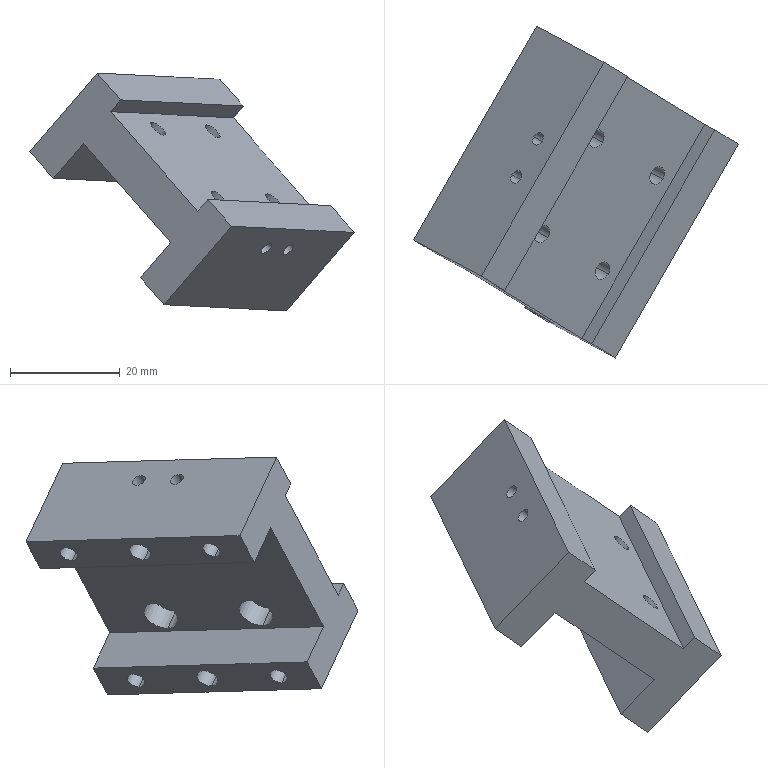Component | SolidWorks | 1z0-123-1 | 1 solid | 74 faces | box 59.17 x 60.52 x 43.37 mm | volume 20475 mm3 | cylinder 36 | cone 20 | plane 18 | commonest cylinder face diameters 2.5 x8 3.3 x8 6.5 x8 3.4 x8 4 x4
build123d program:
from build123d import *

# Parameters (mm, degrees)
SKETCH1_W                                       = 40
SKETCH1_H                                       = 45
BOSS_EXTRUDE1_DEPTH                             = 20
SKETCH2_W                                       = 26
SKETCH2_H                                       = 45
CUT_EXTRUDE1_DEPTH                              = 3
M3_HEX_SOCKET_HEAD_CAP_SCREW_CBORE1_D           = 3.4
M3_HEX_SOCKET_HEAD_CAP_SCREW_CBORE1_CBORE_D     = 6.5
M3_HEX_SOCKET_HEAD_CAP_SCREW_CBORE1_CBORE_DEPTH = 13.4
SKETCH5_W                                       = 26
SKETCH5_H                                       = 18
CUT_EXTRUDE2_DEPTH                              = 54.151
M4_TAPPED_HOLE1_D                               = 3.3
M4_TAPPED_HOLE1_DEPTH                           = 10.1
M4_TAPPED_HOLE1_TIP                             = 0.9914
SIZE_MM_DOWEL_PIN_HOLE1_D                       = 4
SIZE_MM_DOWEL_PIN_HOLE1_DEPTH                   = 10
SIZE_MM_DOWEL_PIN_HOLE1_TIP                     = 1.202
M3_TAPPED_HOLE1_AT_2_COUNT                      = 2
M3_TAPPED_HOLE1_AT_2_PITCH                      = 8


with BuildPart() as part:
    # Sketch1 → Boss-Extrude1 (new body)
    with BuildSketch(Plane.XY):
        Rectangle(SKETCH1_W, SKETCH1_H)
    extrude(amount=BOSS_EXTRUDE1_DEPTH)

    # Sketch2 → Cut-Extrude1 (cut)
    with BuildSketch(Plane(origin=(0, 0, 0), x_dir=(-1, 0, 0), z_dir=(0, 0, -1))):
        Rectangle(SKETCH2_W, SKETCH2_H)
    extrude(amount=-CUT_EXTRUDE1_DEPTH, mode=Mode.SUBTRACT)

    # M3 Hex Socket Head Cap Screw CBORE1 (through all)
    with Locations(Plane(origin=(-9, 10, 20), x_dir=(1, 0, 0), z_dir=(0, 0, 1))):
        with Locations((0, 0), (18, 0), (18, -20), (0, -20)):
            CounterBoreHole(M3_HEX_SOCKET_HEAD_CAP_SCREW_CBORE1_D / 2, M3_HEX_SOCKET_HEAD_CAP_SCREW_CBORE1_CBORE_D / 2, M3_HEX_SOCKET_HEAD_CAP_SCREW_CBORE1_CBORE_DEPTH)

    # Sketch5 → Cut-Extrude2 (cut, through all)
    with BuildSketch(Plane(origin=(0, -22.5, 0), x_dir=(-1, 0, 0), z_dir=(0, -1, 0))):
        with Locations((0, -20)):
            Rectangle(SKETCH5_W, SKETCH5_H)
    extrude(amount=-CUT_EXTRUDE2_DEPTH, mode=Mode.SUBTRACT)

    # M4 Tapped Hole1
    with Locations(Plane(origin=(-16.5, 15, 20), x_dir=(1, 0, 0), z_dir=(0, 0, 1))):
        with Locations((0, 0), (33, 0), (33, -30), (0, -30)):
            Hole(M4_TAPPED_HOLE1_D / 2, depth=M4_TAPPED_HOLE1_DEPTH)
            with Locations((0, 0, -(M4_TAPPED_HOLE1_DEPTH + M4_TAPPED_HOLE1_TIP / 2))):  # 118° drill point
                Cone(0, M4_TAPPED_HOLE1_D / 2, M4_TAPPED_HOLE1_TIP, mode=Mode.SUBTRACT)

    # Size mm Dowel Pin Hole1
    with Locations(Plane(origin=(-16.5, 0, 20), x_dir=(1, 0, 0), z_dir=(0, 0, 1))):
        with Locations((0, 0), (33, 0)):
            Hole(SIZE_MM_DOWEL_PIN_HOLE1_D / 2, depth=SIZE_MM_DOWEL_PIN_HOLE1_DEPTH)
            with Locations((0, 0, -(SIZE_MM_DOWEL_PIN_HOLE1_DEPTH + SIZE_MM_DOWEL_PIN_HOLE1_TIP / 2))):  # 118° drill point
                Cone(0, SIZE_MM_DOWEL_PIN_HOLE1_D / 2, SIZE_MM_DOWEL_PIN_HOLE1_TIP, mode=Mode.SUBTRACT)

    # Sketch9 → M3 Tapped Hole1 (revolve, cut)
    with BuildSketch(Plane(origin=(-20, 4.5, 5), x_dir=(0, 0, 1), z_dir=(0, 1, 0))):
        Polygon((0, 0), (0, 8.251), (1.25, 7.5), (1.25, 0), align=None)
    m3_tapped_hole1 = revolve(axis=Axis((-26.35, 4.5, 5), (1, 0, 0)), mode=Mode.SUBTRACT)

    # M3 Tapped Hole1 at 2: M3 Tapped Hole1 ×2
    with Locations(*[(0, -i * M3_TAPPED_HOLE1_AT_2_PITCH, 0) for i in range(1, M3_TAPPED_HOLE1_AT_2_COUNT)]):
        add(m3_tapped_hole1, mode=Mode.SUBTRACT)

    # Mirror1: M3 Tapped Hole1 across plane
    add(m3_tapped_hole1.mirror(Plane(origin=(0, 0, 0), x_dir=(0, 0, 1), z_dir=(1, 0, 0))), mode=Mode.SUBTRACT)

    # Mirror1 copy 1 sketch → Mirror1 copy 1 (revolve, cut)
    with BuildSketch(Plane(origin=(20, -3.5, 5), x_dir=(0, 0, 1), z_dir=(0, 1, 0))):
        Polygon((0, 0), (0, -8.251), (1.25, -7.5), (1.25, 0), align=None)
    revolve(axis=Axis((26.35, -3.5, 5), (1, 0, 0)), mode=Mode.SUBTRACT)


solid = part.part

# Placed as in the assembly
solid = solid.moved(Location((-14.525, -114.679, 146.305), (-155.101, -37.93, -140.876)))